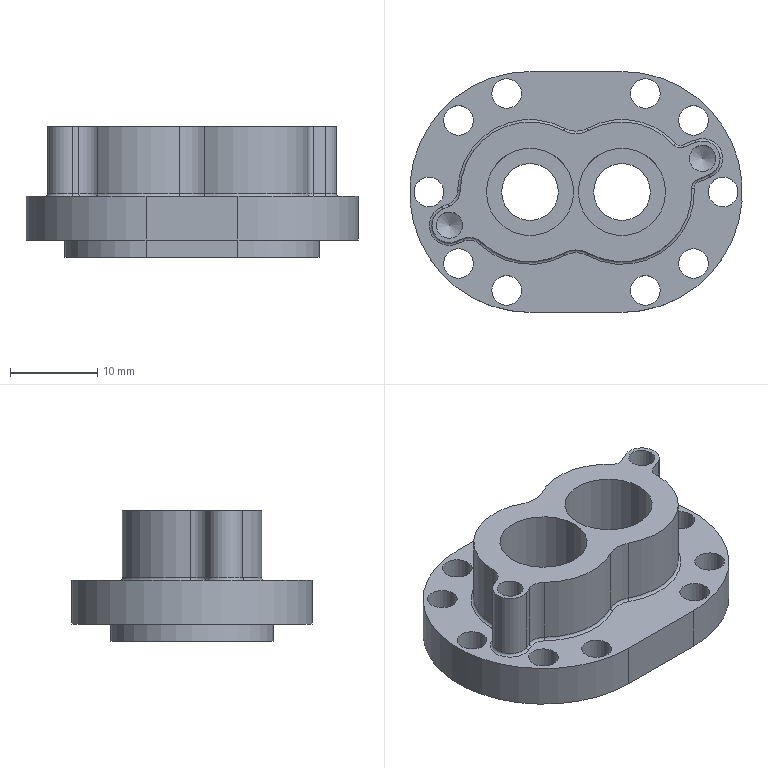Component | NX | FRONT_COVER | 1 solid | 69 faces | volume 5511 mm3 | cylinder 38 | plane 17 | torus 12 | cone 2 | commonest cylinder face diameters 3.4 x10 16 x4 4 x4 0.6 x4 6 x2 10 x2 27.6 x2 6.5 x2